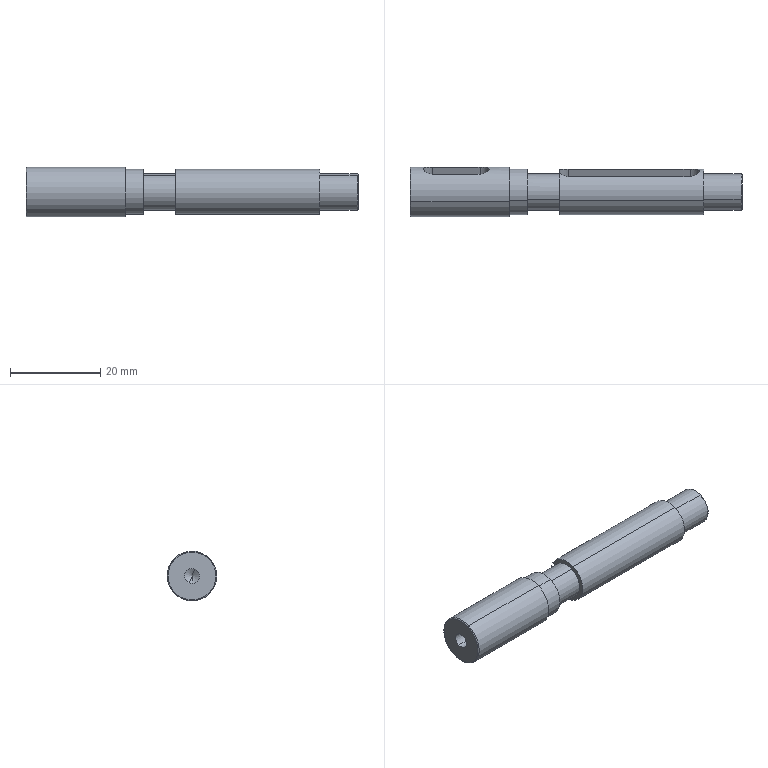Component | SolidWorks | ZHDJ-G004-1 | 1 solid | 38 faces | box 73.5 x 11 x 11 mm | volume 5036 mm3 | cylinder 18 | plane 12 | torus 4 | cone 4 | commonest cylinder face diameters 10 x4 8 x4 3.3 x4 4 x4 11 x2
build123d program:
from build123d import *

# Parameters (mm, degrees)
SKETCH1_2_R                     = 5
BOSS_EXTRUDE1_DEPTH             = 21.5
SKETCH2_R                       = 5.5
BOSS_EXTRUDE2_DEPTH             = 22
CUT_EXTRUDE1_2_DEPTH            = 10
SKETCH5_R                       = 4
BOSS_EXTRUDE3_DEPTH             = 8.5
FILLET1_R                       = 0.2
M4_TAPPED_HOLE1_D               = 3.3
M4_TAPPED_HOLE1_DEPTH           = 11.5
M4_TAPPED_HOLE1_TIP             = 0.9914
M4_TAPPED_HOLE1_ON_FACE_2_D     = 3.3
M4_TAPPED_HOLE1_ON_FACE_2_DEPTH = 11.5
M4_TAPPED_HOLE1_ON_FACE_2_TIP   = 0.9914
CUT_EXTRUDE2_DEPTH              = 10
SKETCH1_R                       = 6
SKETCH1_R_2                     = 4
CUT_EXTRUDE1_DEPTH              = 3.55


with BuildPart() as part:
    # Sketch1_2 → Boss-Extrude1 (new, symmetric)
    with BuildSketch(Plane(origin=(0, 0, 0), x_dir=(0, 0, -1), z_dir=(1, 0, 0))):
        Circle(SKETCH1_2_R)
    extrude(amount=BOSS_EXTRUDE1_DEPTH, both=True)

    # Sketch2 → Boss-Extrude2 (add)
    with BuildSketch(Plane.ZY.offset(21.5)):
        Circle(SKETCH2_R)
    extrude(amount=BOSS_EXTRUDE2_DEPTH)

    # Sketch4 → Cut-Extrude1_2 (cut)
    with BuildSketch(Plane(origin=(0, 2.3, 0), x_dir=(1, 0, 0), z_dir=(0, 1, 0))):
        with BuildLine():
            Line((18.5, -2), (-8.5, -2))
            ThreePointArc((-8.5, -2), (-10.5, 0), (-8.5, 2))
            Line((-8.5, 2), (18.5, 2))
            ThreePointArc((18.5, 2), (20.5, 0), (18.5, -2))
        make_face()
    extrude(amount=CUT_EXTRUDE1_2_DEPTH, mode=Mode.SUBTRACT)

    # Sketch5 → Boss-Extrude3 (add)
    with BuildSketch(Plane(origin=(21.5, 0, 0), x_dir=(0, 0, -1), z_dir=(1, 0, 0))):
        Circle(SKETCH5_R)
    extrude(amount=BOSS_EXTRUDE3_DEPTH)

    # Fillet1
    fillet1_edges = [part.edges().sort_by_distance(p)[0] for p in [
        (30, 0, 4),
        (-43.5, 0, -5.5),
    ]]
    fillet(fillet1_edges, radius=FILLET1_R)

    # M4 Tapped Hole1
    with Locations(Plane(origin=(-43.5, 0, 0), x_dir=(0, 0, -1), z_dir=(-1, 0, 0))):
        with Locations((0, 0)):
            Hole(M4_TAPPED_HOLE1_D / 2, depth=M4_TAPPED_HOLE1_DEPTH)
            with Locations((0, 0, -(M4_TAPPED_HOLE1_DEPTH + M4_TAPPED_HOLE1_TIP / 2))):  # 118° drill point
                Cone(0, M4_TAPPED_HOLE1_D / 2, M4_TAPPED_HOLE1_TIP, mode=Mode.SUBTRACT)

    # M4 Tapped Hole1 on face 2
    with Locations(Plane(origin=(30, 0, 0), x_dir=(0, 0, 1), z_dir=(1, 0, 0))):
        with Locations((0, 0)):
            Hole(M4_TAPPED_HOLE1_ON_FACE_2_D / 2, depth=M4_TAPPED_HOLE1_ON_FACE_2_DEPTH)
            with Locations((0, 0, -(M4_TAPPED_HOLE1_ON_FACE_2_DEPTH + M4_TAPPED_HOLE1_ON_FACE_2_TIP / 2))):  # 118° drill point
                Cone(0, M4_TAPPED_HOLE1_ON_FACE_2_D / 2, M4_TAPPED_HOLE1_ON_FACE_2_TIP, mode=Mode.SUBTRACT)

    # Sketch7 → Cut-Extrude2 (cut)
    with BuildSketch(Plane(origin=(0, 2.7, 0), x_dir=(1, 0, 0), z_dir=(0, 1, 0))):
        with BuildLine():
            Line((-38.5, 2), (-28, 2))
            ThreePointArc((-28, 2), (-26, 0), (-28, -2))
            Line((-28, -2), (-38.5, -2))
            ThreePointArc((-38.5, -2), (-40.5, 0), (-38.5, 2))
        make_face()
    extrude(amount=CUT_EXTRUDE2_DEPTH, mode=Mode.SUBTRACT)

    # Sketch1 → Cut-Extrude1 (cut, symmetric)
    with BuildSketch(Plane(origin=(-13.95, 0, 0), x_dir=(0, 0, -1), z_dir=(1, 0, 0))):
        Circle(SKETCH1_R)
        Circle(SKETCH1_R_2, mode=Mode.SUBTRACT)
    extrude(amount=CUT_EXTRUDE1_DEPTH, both=True, mode=Mode.SUBTRACT)


solid = part.part

# Placed as in the assembly
solid = solid.moved(Location((15.5, 0, 150), (23.487, 0, 0)))